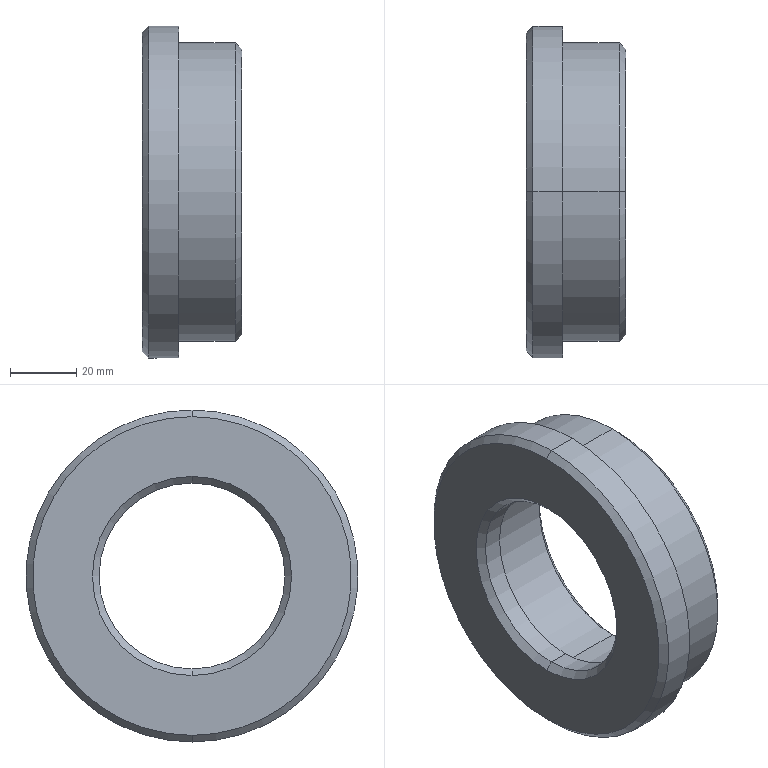Component | SolidWorks | THK-A1005LiftingMotorMountingRoundPlateRight-1 | 1 solid | 20 faces | box 30 x 100 x 100 mm | volume 119208 mm3 | cone 8 | cylinder 8 | plane 4 | commonest cylinder face diameters 56 x2 100 x2 90 x2 62 x2 | material 45
build123d program:
from build123d import *

# Parameters (mm, degrees)
CHAMFER2_SIZE = 2


with BuildPart() as part:
    # Sketch4 → Revolve1 (revolve)
    with BuildSketch(Plane(origin=(0, 0, 0), x_dir=(1, 0, 0), z_dir=(0, 1, 0)), mode=Mode.PRIVATE) as revolve1_sk:
        Polygon((0, 31), (0, 45), (-19, 45), (-19, 50), (-30, 50), (-30, 28), (-22, 28), (-22, 31), align=None)
    revolve(revolve1_sk.sketch.rotate(Axis((-49.996, 0, 0), (1, 0, 0)), 180), axis=Axis((-49.996, 0, 0), (1, 0, 0)))

    # Chamfer2
    chamfer2_edges = [part.edges().sort_by_distance(p)[0] for p in [
        (-30, 0, -28),
        (-30, 0, -50),
        (0, 0, -45),
        (0, 0, -31),
    ]]
    chamfer(chamfer2_edges, length=CHAMFER2_SIZE)


solid = part.part

# Placed as in the assembly
solid = solid.moved(Location((135, 383, -155), (0, 0, 0)))
STEP:
#1=COLOUR_RGB('',0.7922,0.8196,0.9333);
#2=FILL_AREA_STYLE_COLOUR('',#1);
#3=FILL_AREA_STYLE('',(#2));
#4=SURFACE_STYLE_FILL_AREA(#3);
#5=SURFACE_SIDE_STYLE('',(#4));
#6=SURFACE_STYLE_USAGE(.BOTH.,#5);
#7=PRESENTATION_STYLE_ASSIGNMENT((#6));
#8=CARTESIAN_POINT('',(4.134,15.079,-4.213));
#9=VERTEX_POINT('',#8);
#10=CARTESIAN_POINT('',(4.134,15.079,-7.992));
#11=VERTEX_POINT('',#10);
#12=CARTESIAN_POINT('',(4.134,15.079,-6.102));
#13=DIRECTION('',(-1.,0.,0.));
#14=DIRECTION('',(0.,0.,-1.));
#15=AXIS2_PLACEMENT_3D('',#12,#13,#14);
#16=CIRCLE('',#15,1.89);
#17=EDGE_CURVE('',#9,#11,#16,.T.);
#18=ORIENTED_EDGE('',*,*,#17,.F.);
#19=CARTESIAN_POINT('',(4.213,15.079,-4.134));
#20=VERTEX_POINT('',#19);
#21=CARTESIAN_POINT('',(4.134,15.079,-4.213));
#22=DIRECTION('',(0.7071,0.,0.7071));
#23=VECTOR('',#22,39.37);
#24=LINE('',#21,#23);
#25=EDGE_CURVE('',#9,#20,#24,.T.);
#26=ORIENTED_EDGE('',*,*,#25,.T.);
#27=CARTESIAN_POINT('',(4.213,15.079,-8.071));
#28=VERTEX_POINT('',#27);
#29=CARTESIAN_POINT('',(4.213,15.079,-6.102));
#30=DIRECTION('',(1.,0.,0.));
#31=DIRECTION('',(0.,0.,-1.));
#32=AXIS2_PLACEMENT_3D('',#29,#30,#31);
#33=CIRCLE('',#32,1.969);
#34=EDGE_CURVE('',#28,#20,#33,.T.);
#35=ORIENTED_EDGE('',*,*,#34,.F.);
#36=CARTESIAN_POINT('',(4.134,15.079,-7.992));
#37=DIRECTION('',(0.7071,0.,-0.7071));
#38=VECTOR('',#37,39.37);
#39=LINE('',#36,#38);
#40=EDGE_CURVE('',#11,#28,#39,.T.);
#41=ORIENTED_EDGE('',*,*,#40,.F.);
#42=EDGE_LOOP('',(#18,#26,#35,#41));
#43=FACE_OUTER_BOUND('',#42,.T.);
#44=CARTESIAN_POINT('',(4.134,15.079,-6.102));
#45=DIRECTION('',(1.,0.,0.));
#46=DIRECTION('',(0.,0.,-1.));
#47=AXIS2_PLACEMENT_3D('',#44,#45,#46);
#48=CONICAL_SURFACE('',#47,1.89,0.7854);
#49=ADVANCED_FACE('',(#43),#48,.T.);
#50=CARTESIAN_POINT('',(5.236,15.079,-4.882));
#51=VERTEX_POINT('',#50);
#52=CARTESIAN_POINT('',(5.236,15.079,-7.323));
#53=VERTEX_POINT('',#52);
#54=CARTESIAN_POINT('',(5.236,15.079,-6.102));
#55=DIRECTION('',(1.,0.,0.));
#56=DIRECTION('',(0.,0.,1.));
#57=AXIS2_PLACEMENT_3D('',#54,#55,#56);
#58=CIRCLE('',#57,1.22);
#59=EDGE_CURVE('',#51,#53,#58,.T.);
#60=ORIENTED_EDGE('',*,*,#59,.F.);
#61=CARTESIAN_POINT('',(5.315,15.079,-4.803));
#62=VERTEX_POINT('',#61);
#63=CARTESIAN_POINT('',(5.315,15.079,-4.803));
#64=DIRECTION('',(0.7071,0.,0.7071));
#65=VECTOR('',#64,39.37);
#66=LINE('',#63,#65);
#67=EDGE_CURVE('',#51,#62,#66,.T.);
#68=ORIENTED_EDGE('',*,*,#67,.T.);
#69=CARTESIAN_POINT('',(5.315,15.079,-7.402));
#70=VERTEX_POINT('',#69);
#71=CARTESIAN_POINT('',(5.315,15.079,-6.102));
#72=DIRECTION('',(-1.,0.,0.));
#73=DIRECTION('',(0.,0.,1.));
#74=AXIS2_PLACEMENT_3D('',#71,#72,#73);
#75=CIRCLE('',#74,1.299);
#76=EDGE_CURVE('',#70,#62,#75,.T.);
#77=ORIENTED_EDGE('',*,*,#76,.F.);
#78=CARTESIAN_POINT('',(5.315,15.079,-7.402));
#79=DIRECTION('',(0.7071,0.,-0.7071));
#80=VECTOR('',#79,39.37);
#81=LINE('',#78,#80);
#82=EDGE_CURVE('',#53,#70,#81,.T.);
#83=ORIENTED_EDGE('',*,*,#82,.F.);
#84=EDGE_LOOP('',(#60,#68,#77,#83));
#85=FACE_OUTER_BOUND('',#84,.T.);
#86=CARTESIAN_POINT('',(5.315,15.079,-6.102));
#87=DIRECTION('',(1.,0.,0.));
#88=DIRECTION('',(0.,0.,-1.));
#89=AXIS2_PLACEMENT_3D('',#86,#87,#88);
#90=CONICAL_SURFACE('',#89,1.299,0.7854);
#91=ADVANCED_FACE('',(#85),#90,.F.);
#92=CARTESIAN_POINT('',(5.315,15.079,-7.795));
#93=VERTEX_POINT('',#92);
#94=CARTESIAN_POINT('',(5.315,15.079,-4.409));
#95=VERTEX_POINT('',#94);
#96=CARTESIAN_POINT('',(5.315,15.079,-6.102));
#97=DIRECTION('',(1.,0.,0.));
#98=DIRECTION('',(0.,0.,1.));
#99=AXIS2_PLACEMENT_3D('',#96,#97,#98);
#100=CIRCLE('',#99,1.693);
#101=EDGE_CURVE('',#93,#95,#100,.T.);
#102=ORIENTED_EDGE('',*,*,#101,.F.);
#103=CARTESIAN_POINT('',(5.236,15.079,-7.874));
#104=VERTEX_POINT('',#103);
#105=CARTESIAN_POINT('',(5.236,15.079,-7.874));
#106=DIRECTION('',(-0.7071,0.,-0.7071));
#107=VECTOR('',#106,39.37);
#108=LINE('',#105,#107);
#109=EDGE_CURVE('',#93,#104,#108,.T.);
#110=ORIENTED_EDGE('',*,*,#109,.T.);
#111=CARTESIAN_POINT('',(5.236,15.079,-4.331));
#112=VERTEX_POINT('',#111);
#113=CARTESIAN_POINT('',(5.236,15.079,-6.102));
#114=DIRECTION('',(-1.,0.,0.));
#115=DIRECTION('',(0.,0.,1.));
#116=AXIS2_PLACEMENT_3D('',#113,#114,#115);
#117=CIRCLE('',#116,1.772);
#118=EDGE_CURVE('',#112,#104,#117,.T.);
#119=ORIENTED_EDGE('',*,*,#118,.F.);
#120=CARTESIAN_POINT('',(5.236,15.079,-4.331));
#121=DIRECTION('',(-0.7071,0.,0.7071));
#122=VECTOR('',#121,39.37);
#123=LINE('',#120,#122);
#124=EDGE_CURVE('',#95,#112,#123,.T.);
#125=ORIENTED_EDGE('',*,*,#124,.F.);
#126=EDGE_LOOP('',(#102,#110,#119,#125));
#127=FACE_OUTER_BOUND('',#126,.T.);
#128=CARTESIAN_POINT('',(5.236,15.079,-6.102));
#129=DIRECTION('',(-1.,0.,0.));
#130=DIRECTION('',(0.,0.,1.));
#131=AXIS2_PLACEMENT_3D('',#128,#129,#130);
#132=CONICAL_SURFACE('',#131,1.772,0.7854);
#133=ADVANCED_FACE('',(#127),#132,.T.);
#134=CARTESIAN_POINT('',(4.213,15.079,-7.205));
#135=VERTEX_POINT('',#134);
#136=CARTESIAN_POINT('',(4.213,15.079,-5.));
#137=VERTEX_POINT('',#136);
#138=CARTESIAN_POINT('',(4.213,15.079,-6.102));
#139=DIRECTION('',(-1.,0.,0.));
#140=DIRECTION('',(0.,0.,-1.));
#141=AXIS2_PLACEMENT_3D('',#138,#139,#140);
#142=CIRCLE('',#141,1.102);
#143=EDGE_CURVE('',#135,#137,#142,.T.);
#144=ORIENTED_EDGE('',*,*,#143,.F.);
#145=CARTESIAN_POINT('',(4.134,15.079,-7.283));
#146=VERTEX_POINT('',#145);
#147=CARTESIAN_POINT('',(4.213,15.079,-7.205));
#148=DIRECTION('',(-0.7071,0.,-0.7071));
#149=VECTOR('',#148,39.37);
#150=LINE('',#147,#149);
#151=EDGE_CURVE('',#135,#146,#150,.T.);
#152=ORIENTED_EDGE('',*,*,#151,.T.);
#153=CARTESIAN_POINT('',(4.134,15.079,-4.921));
#154=VERTEX_POINT('',#153);
#155=CARTESIAN_POINT('',(4.134,15.079,-6.102));
#156=DIRECTION('',(1.,0.,0.));
#157=DIRECTION('',(0.,0.,-1.));
#158=AXIS2_PLACEMENT_3D('',#155,#156,#157);
#159=CIRCLE('',#158,1.181);
#160=EDGE_CURVE('',#154,#146,#159,.T.);
#161=ORIENTED_EDGE('',*,*,#160,.F.);
#162=CARTESIAN_POINT('',(4.213,15.079,-5.));
#163=DIRECTION('',(-0.7071,0.,0.7071));
#164=VECTOR('',#163,39.37);
#165=LINE('',#162,#164);
#166=EDGE_CURVE('',#137,#154,#165,.T.);
#167=ORIENTED_EDGE('',*,*,#166,.F.);
#168=EDGE_LOOP('',(#144,#152,#161,#167));
#169=FACE_OUTER_BOUND('',#168,.T.);
#170=CARTESIAN_POINT('',(4.213,15.079,-6.102));
#171=DIRECTION('',(-1.,0.,0.));
#172=DIRECTION('',(0.,0.,1.));
#173=AXIS2_PLACEMENT_3D('',#170,#171,#172);
#174=CONICAL_SURFACE('',#173,1.102,0.7854);
#175=ADVANCED_FACE('',(#169),#174,.F.);
#176=CARTESIAN_POINT('',(4.449,15.079,-7.205));
#177=VERTEX_POINT('',#176);
#178=CARTESIAN_POINT('',(4.449,15.079,-5.));
#179=VERTEX_POINT('',#178);
#180=CARTESIAN_POINT('',(4.449,15.079,-6.102));
#181=DIRECTION('',(-1.,0.,0.));
#182=DIRECTION('',(0.,0.,1.));
#183=AXIS2_PLACEMENT_3D('',#180,#181,#182);
#184=CIRCLE('',#183,1.102);
#185=EDGE_CURVE('',#177,#179,#184,.T.);
#186=ORIENTED_EDGE('',*,*,#185,.F.);
#187=CARTESIAN_POINT('',(3.347,15.079,-7.205));
#188=DIRECTION('',(-1.,0.,0.));
#189=VECTOR('',#188,39.37);
#190=LINE('',#187,#189);
#191=EDGE_CURVE('',#177,#135,#190,.T.);
#192=ORIENTED_EDGE('',*,*,#191,.T.);
#193=ORIENTED_EDGE('',*,*,#143,.T.);
#194=CARTESIAN_POINT('',(3.347,15.079,-5.));
#195=DIRECTION('',(-1.,0.,0.));
#196=VECTOR('',#195,39.37);
#197=LINE('',#194,#196);
#198=EDGE_CURVE('',#179,#137,#197,.T.);
#199=ORIENTED_EDGE('',*,*,#198,.F.);
#200=EDGE_LOOP('',(#186,#192,#193,#199));
#201=FACE_OUTER_BOUND('',#200,.T.);
#202=CARTESIAN_POINT('',(3.347,15.079,-6.102));
#203=DIRECTION('',(-1.,0.,0.));
#204=DIRECTION('',(0.,0.,1.));
#205=AXIS2_PLACEMENT_3D('',#202,#203,#204);
#206=CYLINDRICAL_SURFACE('',#205,1.102);
#207=ADVANCED_FACE('',(#201),#206,.F.);
#208=CARTESIAN_POINT('',(4.567,15.079,-4.134));
#209=VERTEX_POINT('',#208);
#210=CARTESIAN_POINT('',(4.567,15.079,-8.071));
#211=VERTEX_POINT('',#210);
#212=CARTESIAN_POINT('',(4.567,15.079,-6.102));
#213=DIRECTION('',(-1.,0.,0.));
#214=DIRECTION('',(0.,0.,1.));
#215=AXIS2_PLACEMENT_3D('',#212,#213,#214);
#216=CIRCLE('',#215,1.969);
#217=EDGE_CURVE('',#209,#211,#216,.T.);
#218=ORIENTED_EDGE('',*,*,#217,.T.);
#219=CARTESIAN_POINT('',(3.347,15.079,-8.071));
#220=DIRECTION('',(-1.,0.,0.));
#221=VECTOR('',#220,39.37);
#222=LINE('',#219,#221);
#223=EDGE_CURVE('',#211,#28,#222,.T.);
#224=ORIENTED_EDGE('',*,*,#223,.T.);
#225=ORIENTED_EDGE('',*,*,#34,.T.);
#226=CARTESIAN_POINT('',(3.347,15.079,-4.134));
#227=DIRECTION('',(-1.,0.,0.));
#228=VECTOR('',#227,39.37);
#229=LINE('',#226,#228);
#230=EDGE_CURVE('',#209,#20,#229,.T.);
#231=ORIENTED_EDGE('',*,*,#230,.F.);
#232=EDGE_LOOP('',(#218,#224,#225,#231));
#233=FACE_OUTER_BOUND('',#232,.T.);
#234=CARTESIAN_POINT('',(3.347,15.079,-6.102));
#235=DIRECTION('',(-1.,0.,0.));
#236=DIRECTION('',(0.,0.,1.));
#237=AXIS2_PLACEMENT_3D('',#234,#235,#236);
#238=CYLINDRICAL_SURFACE('',#237,1.969);
#239=ADVANCED_FACE('',(#233),#238,.T.);
#240=ORIENTED_EDGE('',*,*,#118,.T.);
#241=CARTESIAN_POINT('',(4.567,15.079,-7.874));
#242=VERTEX_POINT('',#241);
#243=CARTESIAN_POINT('',(3.347,15.079,-7.874));
#244=DIRECTION('',(-1.,0.,0.));
#245=VECTOR('',#244,39.37);
#246=LINE('',#243,#245);
#247=EDGE_CURVE('',#104,#242,#246,.T.);
#248=ORIENTED_EDGE('',*,*,#247,.T.);
#249=CARTESIAN_POINT('',(4.567,15.079,-4.331));
#250=VERTEX_POINT('',#249);
#251=CARTESIAN_POINT('',(4.567,15.079,-6.102));
#252=DIRECTION('',(-1.,0.,0.));
#253=DIRECTION('',(0.,0.,1.));
#254=AXIS2_PLACEMENT_3D('',#251,#252,#253);
#255=CIRCLE('',#254,1.772);
#256=EDGE_CURVE('',#250,#242,#255,.T.);
#257=ORIENTED_EDGE('',*,*,#256,.F.);
#258=CARTESIAN_POINT('',(3.347,15.079,-4.331));
#259=DIRECTION('',(-1.,0.,0.));
#260=VECTOR('',#259,39.37);
#261=LINE('',#258,#260);
#262=EDGE_CURVE('',#112,#250,#261,.T.);
#263=ORIENTED_EDGE('',*,*,#262,.F.);
#264=EDGE_LOOP('',(#240,#248,#257,#263));
#265=FACE_OUTER_BOUND('',#264,.T.);
#266=CARTESIAN_POINT('',(3.347,15.079,-6.102));
#267=DIRECTION('',(-1.,0.,0.));
#268=DIRECTION('',(0.,0.,1.));
#269=AXIS2_PLACEMENT_3D('',#266,#267,#268);
#270=CYLINDRICAL_SURFACE('',#269,1.772);
#271=ADVANCED_FACE('',(#265),#270,.T.);
#272=ORIENTED_EDGE('',*,*,#59,.T.);
#273=CARTESIAN_POINT('',(4.449,15.079,-7.323));
#274=VERTEX_POINT('',#273);
#275=CARTESIAN_POINT('',(3.347,15.079,-7.323));
#276=DIRECTION('',(-1.,0.,0.));
#277=VECTOR('',#276,39.37);
#278=LINE('',#275,#277);
#279=EDGE_CURVE('',#53,#274,#278,.T.);
#280=ORIENTED_EDGE('',*,*,#279,.T.);
#281=CARTESIAN_POINT('',(4.449,15.079,-4.882));
#282=VERTEX_POINT('',#281);
#283=CARTESIAN_POINT('',(4.449,15.079,-6.102));
#284=DIRECTION('',(-1.,0.,0.));
#285=DIRECTION('',(0.,0.,1.));
#286=AXIS2_PLACEMENT_3D('',#283,#284,#285);
#287=CIRCLE('',#286,1.22);
#288=EDGE_CURVE('',#274,#282,#287,.T.);
#289=ORIENTED_EDGE('',*,*,#288,.T.);
#290=CARTESIAN_POINT('',(3.347,15.079,-4.882));
#291=DIRECTION('',(-1.,0.,0.));
#292=VECTOR('',#291,39.37);
#293=LINE('',#290,#292);
#294=EDGE_CURVE('',#51,#282,#293,.T.);
#295=ORIENTED_EDGE('',*,*,#294,.F.);
#296=EDGE_LOOP('',(#272,#280,#289,#295));
#297=FACE_OUTER_BOUND('',#296,.T.);
#298=CARTESIAN_POINT('',(3.347,15.079,-6.102));
#299=DIRECTION('',(-1.,0.,0.));
#300=DIRECTION('',(0.,0.,1.));
#301=AXIS2_PLACEMENT_3D('',#298,#299,#300);
#302=CYLINDRICAL_SURFACE('',#301,1.22);
#303=ADVANCED_FACE('',(#297),#302,.F.);
#304=ORIENTED_EDGE('',*,*,#279,.F.);
#305=CARTESIAN_POINT('',(5.236,15.079,-6.102));
#306=DIRECTION('',(1.,0.,0.));
#307=DIRECTION('',(0.,0.,1.));
#308=AXIS2_PLACEMENT_3D('',#305,#306,#307);
#309=CIRCLE('',#308,1.22);
#310=EDGE_CURVE('',#53,#51,#309,.T.);
#311=ORIENTED_EDGE('',*,*,#310,.T.);
#312=ORIENTED_EDGE('',*,*,#294,.T.);
#313=CARTESIAN_POINT('',(4.449,15.079,-6.102));
#314=DIRECTION('',(-1.,0.,0.));
#315=DIRECTION('',(0.,0.,1.));
#316=AXIS2_PLACEMENT_3D('',#313,#314,#315);
#317=CIRCLE('',#316,1.22);
#318=EDGE_CURVE('',#282,#274,#317,.T.);
#319=ORIENTED_EDGE('',*,*,#318,.T.);
#320=EDGE_LOOP('',(#304,#311,#312,#319));
#321=FACE_OUTER_BOUND('',#320,.T.);
#322=CARTESIAN_POINT('',(3.347,15.079,-6.102));
#323=DIRECTION('',(-1.,0.,0.));
#324=DIRECTION('',(0.,0.,1.));
#325=AXIS2_PLACEMENT_3D('',#322,#323,#324);
#326=CYLINDRICAL_SURFACE('',#325,1.22);
#327=ADVANCED_FACE('',(#321),#326,.F.);
#328=CARTESIAN_POINT('',(5.315,15.079,-6.102));
#329=DIRECTION('',(1.,0.,0.));
#330=DIRECTION('',(0.,0.,1.));
#331=AXIS2_PLACEMENT_3D('',#328,#329,#330);
#332=CIRCLE('',#331,1.693);
#333=EDGE_CURVE('',#95,#93,#332,.T.);
#334=ORIENTED_EDGE('',*,*,#333,.T.);
#335=ORIENTED_EDGE('',*,*,#101,.T.);
#336=EDGE_LOOP('',(#334,#335));
#337=FACE_OUTER_BOUND('',#336,.T.);
#338=ORIENTED_EDGE('',*,*,#76,.T.);
#339=CARTESIAN_POINT('',(5.315,15.079,-6.102));
#340=DIRECTION('',(-1.,0.,0.));
#341=DIRECTION('',(0.,0.,1.));
#342=AXIS2_PLACEMENT_3D('',#339,#340,#341);
#343=CIRCLE('',#342,1.299);
#344=EDGE_CURVE('',#62,#70,#343,.T.);
#345=ORIENTED_EDGE('',*,*,#344,.T.);
#346=EDGE_LOOP('',(#338,#345));
#347=FACE_BOUND('',#346,.T.);
#348=CARTESIAN_POINT('',(5.315,15.079,-7.323));
#349=DIRECTION('',(-1.,0.,0.));
#350=DIRECTION('',(0.,0.,1.));
#351=AXIS2_PLACEMENT_3D('',#348,#349,#350);
#352=PLANE('',#351);
#353=ADVANCED_FACE('',(#337,#347),#352,.F.);
#354=ORIENTED_EDGE('',*,*,#247,.F.);
#355=CARTESIAN_POINT('',(5.236,15.079,-6.102));
#356=DIRECTION('',(-1.,0.,0.));
#357=DIRECTION('',(0.,0.,1.));
#358=AXIS2_PLACEMENT_3D('',#355,#356,#357);
#359=CIRCLE('',#358,1.772);
#360=EDGE_CURVE('',#104,#112,#359,.T.);
#361=ORIENTED_EDGE('',*,*,#360,.T.);
#362=ORIENTED_EDGE('',*,*,#262,.T.);
#363=CARTESIAN_POINT('',(4.567,15.079,-6.102));
#364=DIRECTION('',(-1.,0.,0.));
#365=DIRECTION('',(0.,0.,1.));
#366=AXIS2_PLACEMENT_3D('',#363,#364,#365);
#367=CIRCLE('',#366,1.772);
#368=EDGE_CURVE('',#242,#250,#367,.T.);
#369=ORIENTED_EDGE('',*,*,#368,.F.);
#370=EDGE_LOOP('',(#354,#361,#362,#369));
#371=FACE_OUTER_BOUND('',#370,.T.);
#372=CARTESIAN_POINT('',(3.347,15.079,-6.102));
#373=DIRECTION('',(-1.,0.,0.));
#374=DIRECTION('',(0.,0.,1.));
#375=AXIS2_PLACEMENT_3D('',#372,#373,#374);
#376=CYLINDRICAL_SURFACE('',#375,1.772);
#377=ADVANCED_FACE('',(#371),#376,.T.);
#378=ORIENTED_EDGE('',*,*,#217,.F.);
#379=CARTESIAN_POINT('',(4.567,15.079,-6.102));
#380=DIRECTION('',(-1.,0.,0.));
#381=DIRECTION('',(0.,0.,1.));
#382=AXIS2_PLACEMENT_3D('',#379,#380,#381);
#383=CIRCLE('',#382,1.969);
#384=EDGE_CURVE('',#211,#209,#383,.T.);
#385=ORIENTED_EDGE('',*,*,#384,.F.);
#386=EDGE_LOOP('',(#378,#385));
#387=FACE_OUTER_BOUND('',#386,.T.);
#388=ORIENTED_EDGE('',*,*,#256,.T.);
#389=ORIENTED_EDGE('',*,*,#368,.T.);
#390=EDGE_LOOP('',(#388,#389));
#391=FACE_BOUND('',#390,.T.);
#392=CARTESIAN_POINT('',(4.567,15.079,-8.071));
#393=DIRECTION('',(-1.,0.,0.));
#394=DIRECTION('',(0.,0.,1.));
#395=AXIS2_PLACEMENT_3D('',#392,#393,#394);
#396=PLANE('',#395);
#397=ADVANCED_FACE('',(#387,#391),#396,.F.);
#398=ORIENTED_EDGE('',*,*,#223,.F.);
#399=ORIENTED_EDGE('',*,*,#384,.T.);
#400=ORIENTED_EDGE('',*,*,#230,.T.);
#401=CARTESIAN_POINT('',(4.213,15.079,-6.102));
#402=DIRECTION('',(1.,0.,0.));
#403=DIRECTION('',(0.,0.,-1.));
#404=AXIS2_PLACEMENT_3D('',#401,#402,#403);
#405=CIRCLE('',#404,1.969);
#406=EDGE_CURVE('',#20,#28,#405,.T.);
#407=ORIENTED_EDGE('',*,*,#406,.T.);
#408=EDGE_LOOP('',(#398,#399,#400,#407));
#409=FACE_OUTER_BOUND('',#408,.T.);
#410=CARTESIAN_POINT('',(3.347,15.079,-6.102));
#411=DIRECTION('',(-1.,0.,0.));
#412=DIRECTION('',(0.,0.,1.));
#413=AXIS2_PLACEMENT_3D('',#410,#411,#412);
#414=CYLINDRICAL_SURFACE('',#413,1.969);
#415=ADVANCED_FACE('',(#409),#414,.T.);
#416=ORIENTED_EDGE('',*,*,#160,.T.);
#417=CARTESIAN_POINT('',(4.134,15.079,-6.102));
#418=DIRECTION('',(1.,0.,0.));
#419=DIRECTION('',(0.,0.,-1.));
#420=AXIS2_PLACEMENT_3D('',#417,#418,#419);
#421=CIRCLE('',#420,1.181);
#422=EDGE_CURVE('',#146,#154,#421,.T.);
#423=ORIENTED_EDGE('',*,*,#422,.T.);
#424=EDGE_LOOP('',(#416,#423));
#425=FACE_BOUND('',#424,.T.);
#426=CARTESIAN_POINT('',(4.134,15.079,-6.102));
#427=DIRECTION('',(-1.,0.,0.));
#428=DIRECTION('',(0.,0.,-1.));
#429=AXIS2_PLACEMENT_3D('',#426,#427,#428);
#430=CIRCLE('',#429,1.89);
#431=EDGE_CURVE('',#11,#9,#430,.T.);
#432=ORIENTED_EDGE('',*,*,#431,.T.);
#433=ORIENTED_EDGE('',*,*,#17,.T.);
#434=EDGE_LOOP('',(#432,#433));
#435=FACE_OUTER_BOUND('',#434,.T.);
#436=CARTESIAN_POINT('',(4.134,15.079,-8.071));
#437=DIRECTION('',(1.,0.,0.));
#438=DIRECTION('',(0.,0.,-1.));
#439=AXIS2_PLACEMENT_3D('',#436,#437,#438);
#440=PLANE('',#439);
#441=ADVANCED_FACE('',(#425,#435),#440,.F.);
#442=ORIENTED_EDGE('',*,*,#191,.F.);
#443=CARTESIAN_POINT('',(4.449,15.079,-6.102));
#444=DIRECTION('',(-1.,0.,0.));
#445=DIRECTION('',(0.,0.,1.));
#446=AXIS2_PLACEMENT_3D('',#443,#444,#445);
#447=CIRCLE('',#446,1.102);
#448=EDGE_CURVE('',#179,#177,#447,.T.);
#449=ORIENTED_EDGE('',*,*,#448,.F.);
#450=ORIENTED_EDGE('',*,*,#198,.T.);
#451=CARTESIAN_POINT('',(4.213,15.079,-6.102));
#452=DIRECTION('',(-1.,0.,0.));
#453=DIRECTION('',(0.,0.,-1.));
#454=AXIS2_PLACEMENT_3D('',#451,#452,#453);
#455=CIRCLE('',#454,1.102);
#456=EDGE_CURVE('',#137,#135,#455,.T.);
#457=ORIENTED_EDGE('',*,*,#456,.T.);
#458=EDGE_LOOP('',(#442,#449,#450,#457));
#459=FACE_OUTER_BOUND('',#458,.T.);
#460=CARTESIAN_POINT('',(3.347,15.079,-6.102));
#461=DIRECTION('',(-1.,0.,0.));
#462=DIRECTION('',(0.,0.,1.));
#463=AXIS2_PLACEMENT_3D('',#460,#461,#462);
#464=CYLINDRICAL_SURFACE('',#463,1.102);
#465=ADVANCED_FACE('',(#459),#464,.F.);
#466=ORIENTED_EDGE('',*,*,#318,.F.);
#467=ORIENTED_EDGE('',*,*,#288,.F.);
#468=EDGE_LOOP('',(#466,#467));
#469=FACE_OUTER_BOUND('',#468,.T.);
#470=ORIENTED_EDGE('',*,*,#448,.T.);
#471=ORIENTED_EDGE('',*,*,#185,.T.);
#472=EDGE_LOOP('',(#470,#471));
#473=FACE_BOUND('',#472,.T.);
#474=CARTESIAN_POINT('',(4.449,15.079,-7.205));
#475=DIRECTION('',(-1.,0.,0.));
#476=DIRECTION('',(0.,0.,1.));
#477=AXIS2_PLACEMENT_3D('',#474,#475,#476);
#478=PLANE('',#477);
#479=ADVANCED_FACE('',(#469,#473),#478,.F.);
#480=ORIENTED_EDGE('',*,*,#151,.F.);
#481=ORIENTED_EDGE('',*,*,#456,.F.);
#482=ORIENTED_EDGE('',*,*,#166,.T.);
#483=ORIENTED_EDGE('',*,*,#422,.F.);
#484=EDGE_LOOP('',(#480,#481,#482,#483));
#485=FACE_OUTER_BOUND('',#484,.T.);
#486=CARTESIAN_POINT('',(4.213,15.079,-6.102));
#487=DIRECTION('',(-1.,0.,0.));
#488=DIRECTION('',(0.,0.,1.));
#489=AXIS2_PLACEMENT_3D('',#486,#487,#488);
#490=CONICAL_SURFACE('',#489,1.102,0.7854);
#491=ADVANCED_FACE('',(#485),#490,.F.);
#492=ORIENTED_EDGE('',*,*,#109,.F.);
#493=ORIENTED_EDGE('',*,*,#333,.F.);
#494=ORIENTED_EDGE('',*,*,#124,.T.);
#495=ORIENTED_EDGE('',*,*,#360,.F.);
#496=EDGE_LOOP('',(#492,#493,#494,#495));
#497=FACE_OUTER_BOUND('',#496,.T.);
#498=CARTESIAN_POINT('',(5.236,15.079,-6.102));
#499=DIRECTION('',(-1.,0.,0.));
#500=DIRECTION('',(0.,0.,1.));
#501=AXIS2_PLACEMENT_3D('',#498,#499,#500);
#502=CONICAL_SURFACE('',#501,1.772,0.7854);
#503=ADVANCED_FACE('',(#497),#502,.T.);
#504=ORIENTED_EDGE('',*,*,#67,.F.);
#505=ORIENTED_EDGE('',*,*,#310,.F.);
#506=ORIENTED_EDGE('',*,*,#82,.T.);
#507=ORIENTED_EDGE('',*,*,#344,.F.);
#508=EDGE_LOOP('',(#504,#505,#506,#507));
#509=FACE_OUTER_BOUND('',#508,.T.);
#510=CARTESIAN_POINT('',(5.315,15.079,-6.102));
#511=DIRECTION('',(1.,0.,0.));
#512=DIRECTION('',(0.,0.,-1.));
#513=AXIS2_PLACEMENT_3D('',#510,#511,#512);
#514=CONICAL_SURFACE('',#513,1.299,0.7854);
#515=ADVANCED_FACE('',(#509),#514,.F.);
#516=ORIENTED_EDGE('',*,*,#25,.F.);
#517=ORIENTED_EDGE('',*,*,#431,.F.);
#518=ORIENTED_EDGE('',*,*,#40,.T.);
#519=ORIENTED_EDGE('',*,*,#406,.F.);
#520=EDGE_LOOP('',(#516,#517,#518,#519));
#521=FACE_OUTER_BOUND('',#520,.T.);
#522=CARTESIAN_POINT('',(4.134,15.079,-6.102));
#523=DIRECTION('',(1.,0.,0.));
#524=DIRECTION('',(0.,0.,-1.));
#525=AXIS2_PLACEMENT_3D('',#522,#523,#524);
#526=CONICAL_SURFACE('',#525,1.89,0.7854);
#527=ADVANCED_FACE('',(#521),#526,.T.);
#528=CLOSED_SHELL('',(#49,#91,#133,#175,#207,#239,#271,#303,#327,#353,#377,#397,#415,#441,#465,#479,#491,#503,#515,#527));
#529=MANIFOLD_SOLID_BREP('',#528);
#530=STYLED_ITEM('',(#7),#529);
#531=(LENGTH_UNIT()NAMED_UNIT(*)SI_UNIT($,.METRE.));
#532=LENGTH_MEASURE_WITH_UNIT(LENGTH_MEASURE(0.0254),#531);
#533=DIMENSIONAL_EXPONENTS(1.,0.,0.,0.,0.,0.,0.);
#534=(CONVERSION_BASED_UNIT('',#532)LENGTH_UNIT()NAMED_UNIT(#533));
#535=UNCERTAINTY_MEASURE_WITH_UNIT(LENGTH_MEASURE(0.00001),#534,'','');
#536=(NAMED_UNIT(*)PLANE_ANGLE_UNIT()SI_UNIT($,.RADIAN.));
#537=(NAMED_UNIT(*)SI_UNIT($,.STERADIAN.)SOLID_ANGLE_UNIT());
#538=(GEOMETRIC_REPRESENTATION_CONTEXT(3)GLOBAL_UNCERTAINTY_ASSIGNED_CONTEXT((#535))GLOBAL_UNIT_ASSIGNED_CONTEXT((#534,#536,#537))REPRESENTATION_CONTEXT('',''));
#539=MECHANICAL_DESIGN_GEOMETRIC_PRESENTATION_REPRESENTATION('',(#530),#538);
#540=PRESENTATION_LAYER_ASSIGNMENT('','',(#530));
#541=CARTESIAN_POINT('',(0.,0.,0.));
#542=DIRECTION('',(0.,0.,1.));
#543=DIRECTION('',(1.,0.,0.));
#544=AXIS2_PLACEMENT_3D('',#541,#542,#543);
#545=(LENGTH_UNIT()NAMED_UNIT(*)SI_UNIT($,.METRE.));
#546=LENGTH_MEASURE_WITH_UNIT(LENGTH_MEASURE(0.0254),#545);
#547=DIMENSIONAL_EXPONENTS(1.,0.,0.,0.,0.,0.,0.);
#548=(CONVERSION_BASED_UNIT('',#546)LENGTH_UNIT()NAMED_UNIT(#547));
#549=UNCERTAINTY_MEASURE_WITH_UNIT(LENGTH_MEASURE(0.00001),#548,'','');
#550=(NAMED_UNIT(*)PLANE_ANGLE_UNIT()SI_UNIT($,.RADIAN.));
#551=(NAMED_UNIT(*)SI_UNIT($,.STERADIAN.)SOLID_ANGLE_UNIT());
#552=(GEOMETRIC_REPRESENTATION_CONTEXT(3)GLOBAL_UNCERTAINTY_ASSIGNED_CONTEXT((#549))GLOBAL_UNIT_ASSIGNED_CONTEXT((#548,#550,#551))REPRESENTATION_CONTEXT('',''));
#553=ADVANCED_BREP_SHAPE_REPRESENTATION('',(#529,#544),#552);